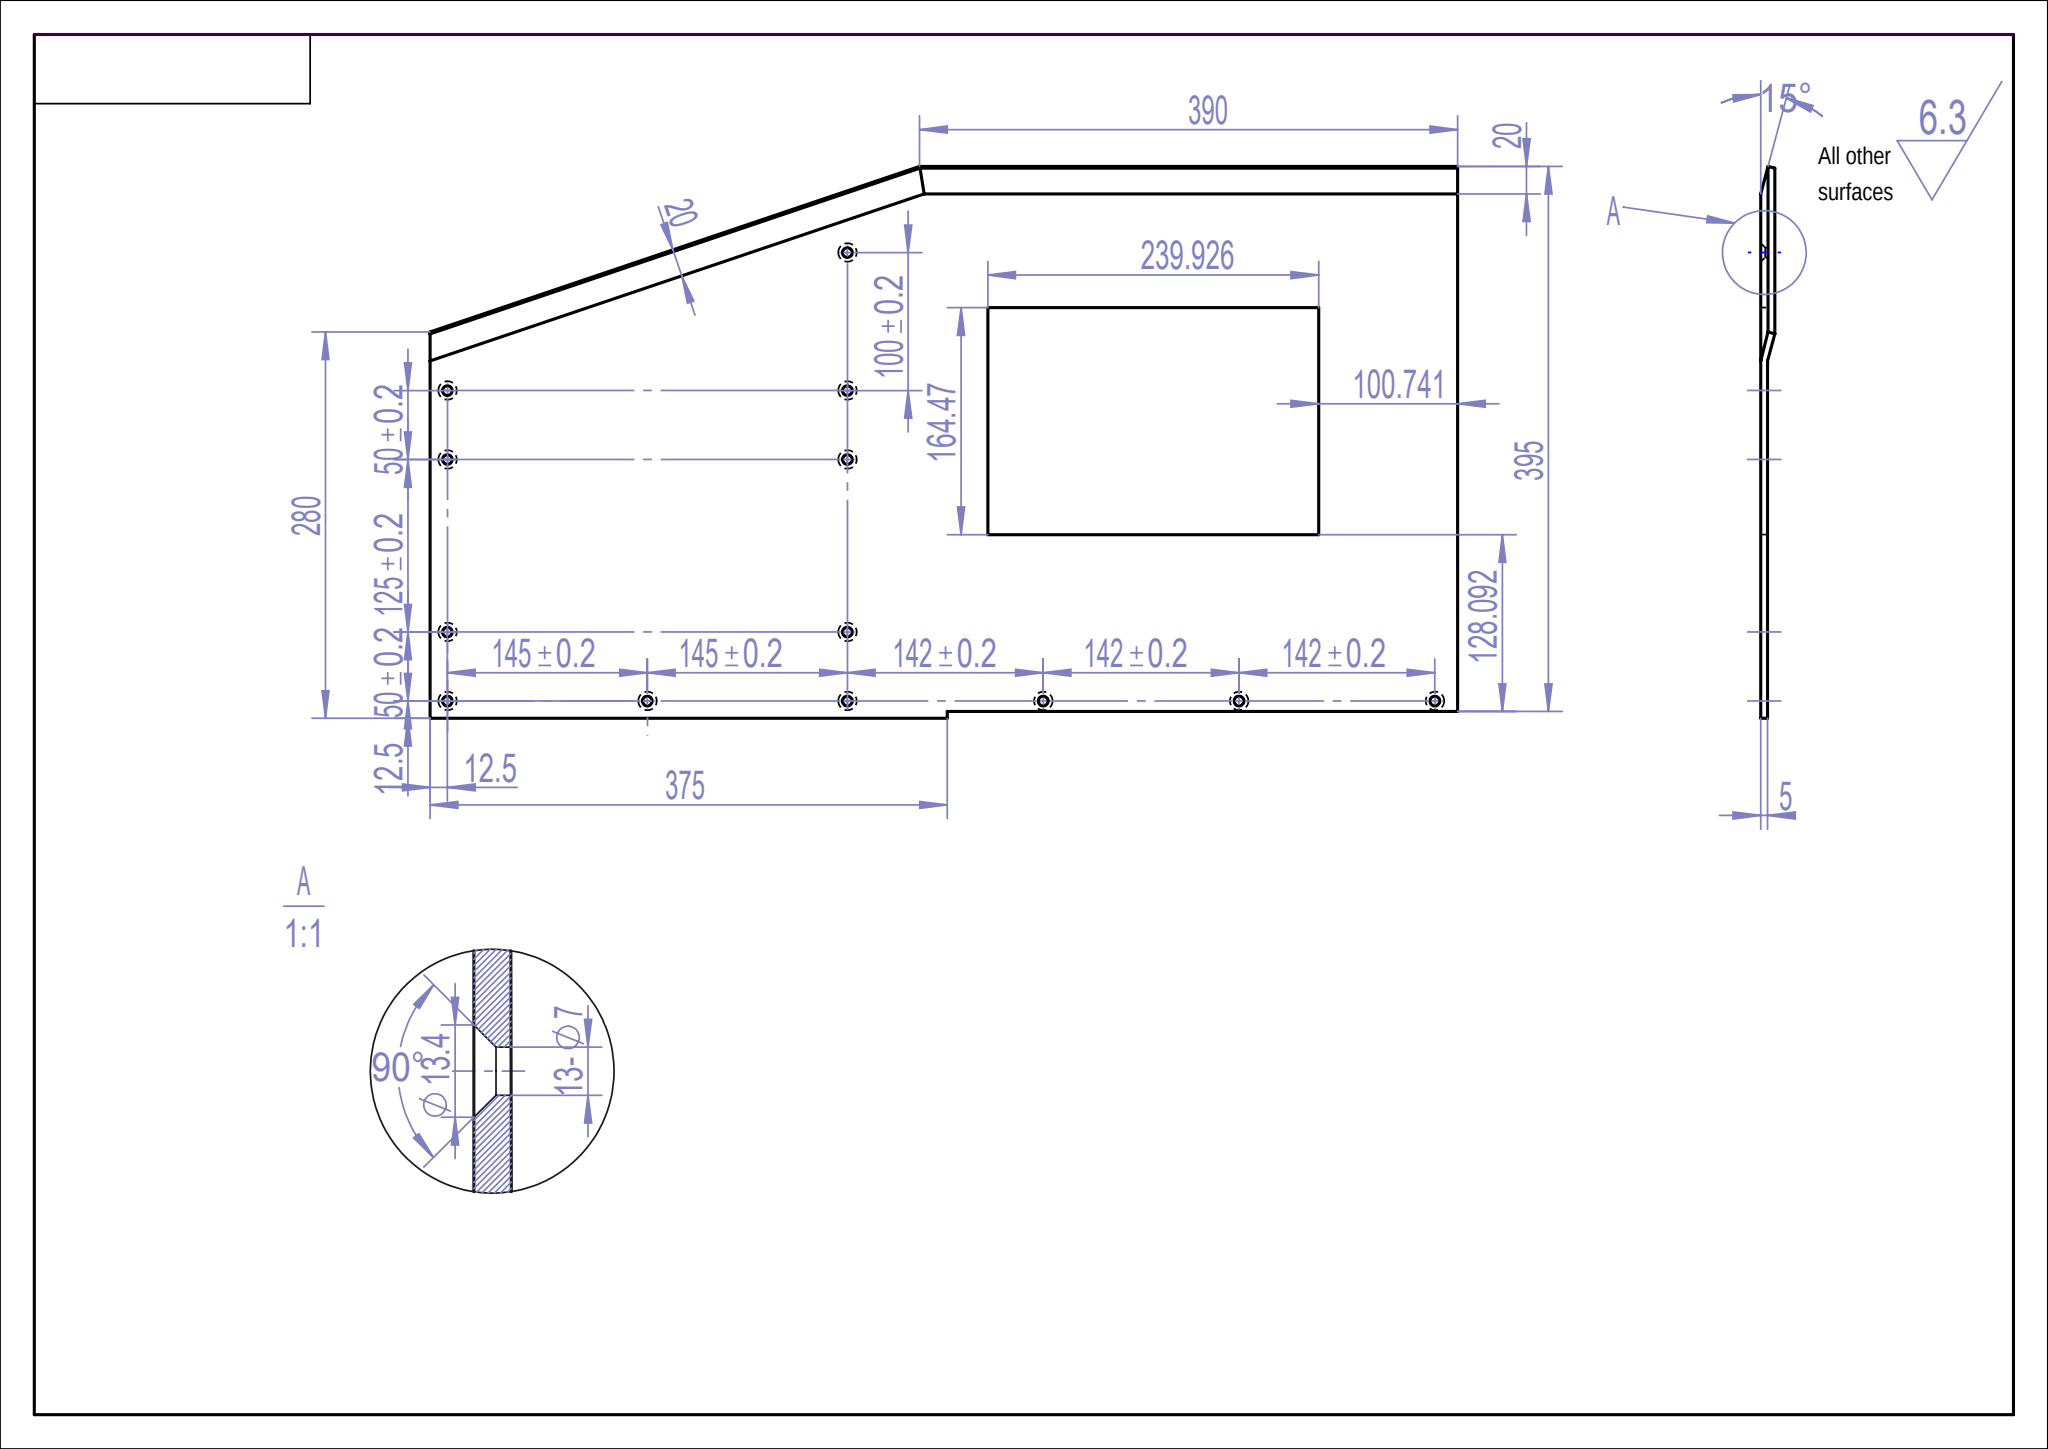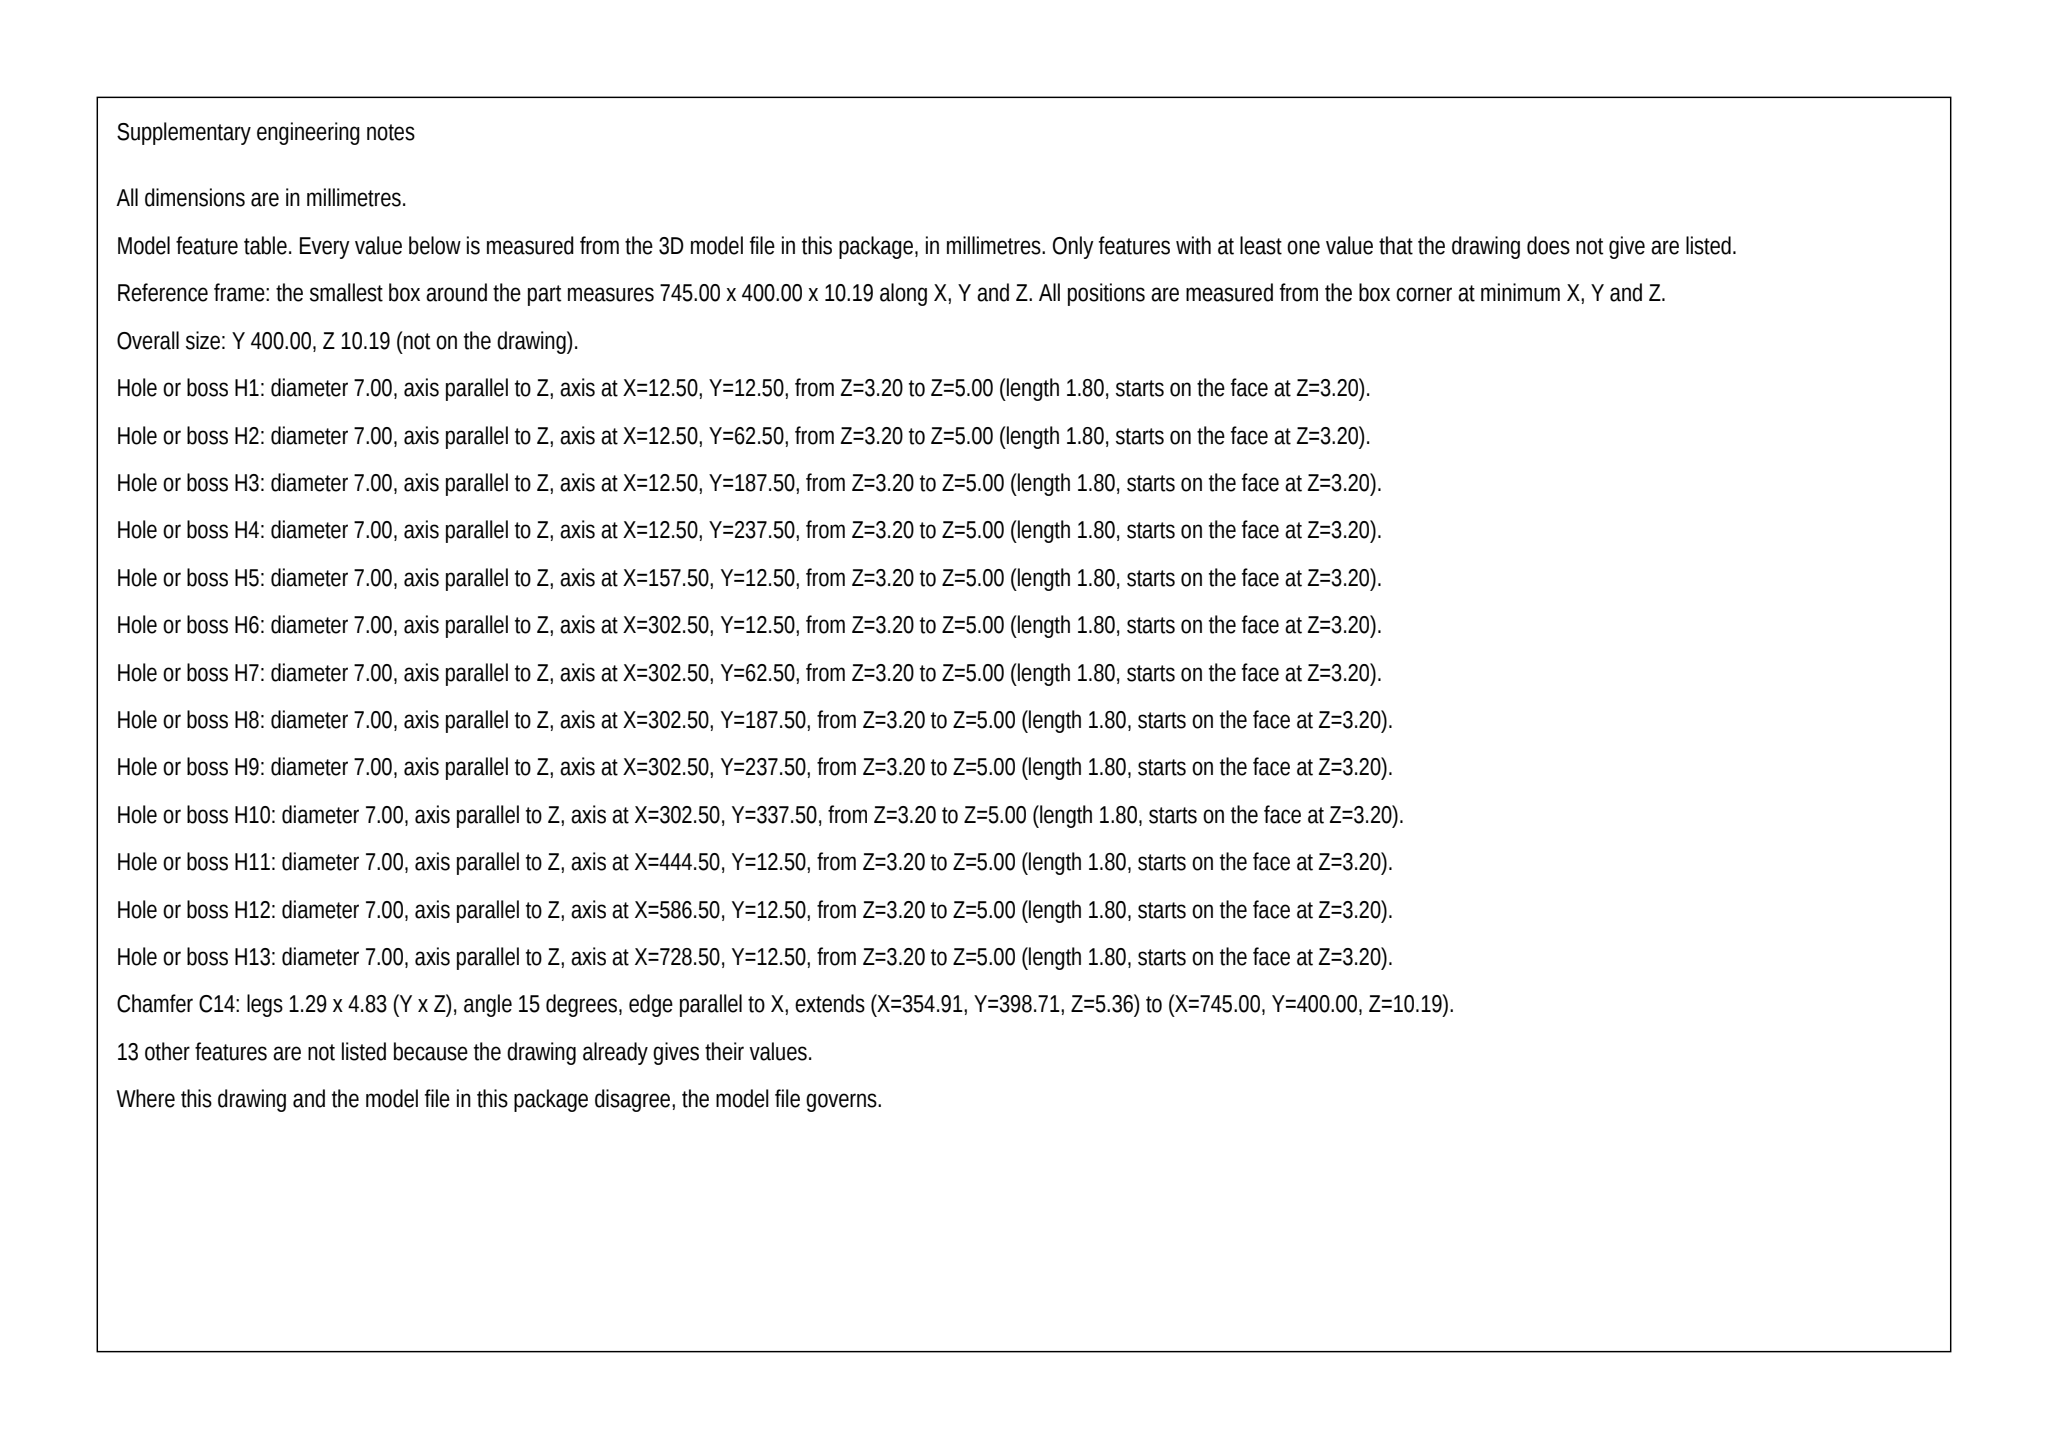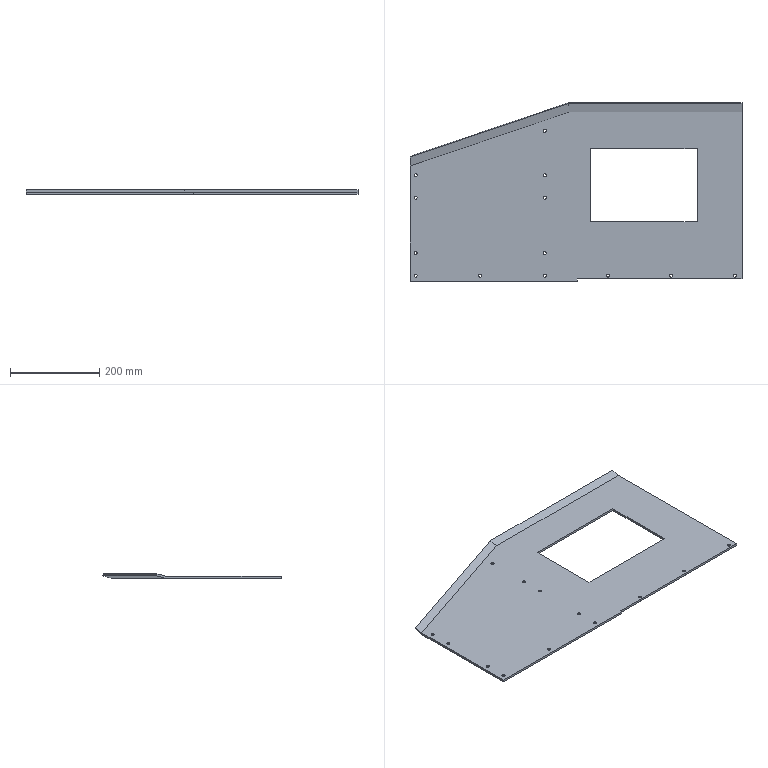Part | SolidWorks | mm | 1 solid | 69 faces | box 745 x 400 x 10.19 mm | volume 1171447 mm3 | cylinder 26 | cone 26 | plane 17 | commonest cylinder face diameters 7 x26